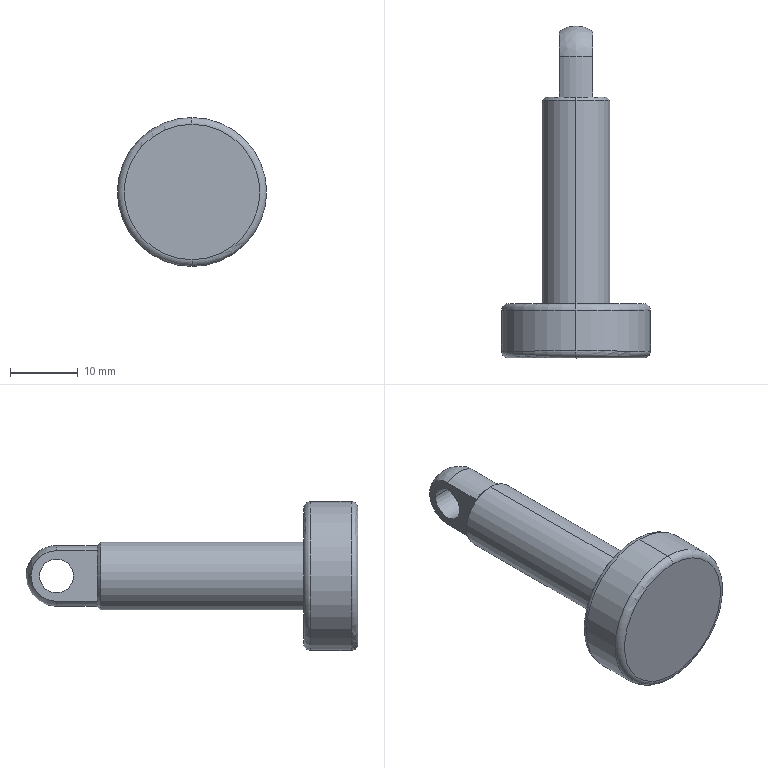Component | SolidWorks | LeverHydraulicRod22-6_HLKA-22_2-1 | 1 solid | 22 faces | box 22 x 49 x 22 mm | volume 5704 mm3 | cylinder 9 | plane 6 | torus 4 | cone 2 | sphere 1 | commonest cylinder face diameters 9 x3 22 x2 5 x2 10 x2
STEP:
#1=COLOUR_RGB('',0.7922,0.8196,0.9333);
#2=FILL_AREA_STYLE_COLOUR('',#1);
#3=FILL_AREA_STYLE('',(#2));
#4=SURFACE_STYLE_FILL_AREA(#3);
#5=SURFACE_SIDE_STYLE('',(#4));
#6=SURFACE_STYLE_USAGE(.BOTH.,#5);
#7=PRESENTATION_STYLE_ASSIGNMENT((#6));
#8=CARTESIAN_POINT('',(-2.662,2.758,4.055));
#9=VERTEX_POINT('',#8);
#10=CARTESIAN_POINT('',(-2.662,2.758,3.189));
#11=VERTEX_POINT('',#10);
#12=CARTESIAN_POINT('',(-2.662,2.758,3.622));
#13=DIRECTION('',(-0.,1.,0.));
#14=DIRECTION('',(0.,0.,-1.));
#15=AXIS2_PLACEMENT_3D('',#12,#13,#14);
#16=CIRCLE('',#15,0.4331);
#17=EDGE_CURVE('',#9,#11,#16,.T.);
#18=ORIENTED_EDGE('',*,*,#17,.F.);
#19=CARTESIAN_POINT('',(-2.662,2.718,4.016));
#20=VERTEX_POINT('',#19);
#21=CARTESIAN_POINT('',(-2.662,2.758,4.016));
#22=DIRECTION('',(1.,0.,0.));
#23=DIRECTION('',(0.,0.,-1.));
#24=AXIS2_PLACEMENT_3D('',#21,#22,#23);
#25=CIRCLE('',#24,0.03937);
#26=EDGE_CURVE('',#9,#20,#25,.T.);
#27=ORIENTED_EDGE('',*,*,#26,.T.);
#28=CARTESIAN_POINT('',(-2.662,2.718,3.228));
#29=VERTEX_POINT('',#28);
#30=CARTESIAN_POINT('',(-2.662,2.718,3.622));
#31=DIRECTION('',(0.,-1.,-0.));
#32=DIRECTION('',(0.,0.,-1.));
#33=AXIS2_PLACEMENT_3D('',#30,#31,#32);
#34=CIRCLE('',#33,0.3937);
#35=EDGE_CURVE('',#29,#20,#34,.T.);
#36=ORIENTED_EDGE('',*,*,#35,.F.);
#37=CARTESIAN_POINT('',(-2.662,2.758,3.228));
#38=DIRECTION('',(-1.,-0.,-0.));
#39=DIRECTION('',(0.,0.,1.));
#40=AXIS2_PLACEMENT_3D('',#37,#38,#39);
#41=CIRCLE('',#40,0.03937);
#42=EDGE_CURVE('',#11,#29,#41,.T.);
#43=ORIENTED_EDGE('',*,*,#42,.F.);
#44=EDGE_LOOP('',(#18,#27,#36,#43));
#45=FACE_OUTER_BOUND('',#44,.T.);
#46=CARTESIAN_POINT('',(-2.662,2.758,3.622));
#47=DIRECTION('',(0.,-1.,-0.));
#48=DIRECTION('',(0.,0.,-1.));
#49=AXIS2_PLACEMENT_3D('',#46,#47,#48);
#50=TOROIDAL_SURFACE('',#49,0.3937,0.03937);
#51=ADVANCED_FACE('',(#45),#50,.T.);
#52=CARTESIAN_POINT('',(-2.662,3.033,4.016));
#53=VERTEX_POINT('',#52);
#54=CARTESIAN_POINT('',(-2.662,3.033,3.228));
#55=VERTEX_POINT('',#54);
#56=CARTESIAN_POINT('',(-2.662,3.033,3.622));
#57=DIRECTION('',(-0.,1.,0.));
#58=DIRECTION('',(0.,0.,-1.));
#59=AXIS2_PLACEMENT_3D('',#56,#57,#58);
#60=CIRCLE('',#59,0.3937);
#61=EDGE_CURVE('',#53,#55,#60,.T.);
#62=ORIENTED_EDGE('',*,*,#61,.F.);
#63=CARTESIAN_POINT('',(-2.662,2.994,4.055));
#64=VERTEX_POINT('',#63);
#65=CARTESIAN_POINT('',(-2.662,2.994,4.016));
#66=DIRECTION('',(1.,0.,0.));
#67=DIRECTION('',(0.,0.,-1.));
#68=AXIS2_PLACEMENT_3D('',#65,#66,#67);
#69=CIRCLE('',#68,0.03937);
#70=EDGE_CURVE('',#53,#64,#69,.T.);
#71=ORIENTED_EDGE('',*,*,#70,.T.);
#72=CARTESIAN_POINT('',(-2.662,2.994,3.189));
#73=VERTEX_POINT('',#72);
#74=CARTESIAN_POINT('',(-2.662,2.994,3.622));
#75=DIRECTION('',(0.,-1.,-0.));
#76=DIRECTION('',(0.,0.,-1.));
#77=AXIS2_PLACEMENT_3D('',#74,#75,#76);
#78=CIRCLE('',#77,0.4331);
#79=EDGE_CURVE('',#73,#64,#78,.T.);
#80=ORIENTED_EDGE('',*,*,#79,.F.);
#81=CARTESIAN_POINT('',(-2.662,2.994,3.228));
#82=DIRECTION('',(-1.,-0.,-0.));
#83=DIRECTION('',(0.,0.,1.));
#84=AXIS2_PLACEMENT_3D('',#81,#82,#83);
#85=CIRCLE('',#84,0.03937);
#86=EDGE_CURVE('',#55,#73,#85,.T.);
#87=ORIENTED_EDGE('',*,*,#86,.F.);
#88=EDGE_LOOP('',(#62,#71,#80,#87));
#89=FACE_OUTER_BOUND('',#88,.T.);
#90=CARTESIAN_POINT('',(-2.662,2.994,3.622));
#91=DIRECTION('',(0.,-1.,-0.));
#92=DIRECTION('',(0.,0.,-1.));
#93=AXIS2_PLACEMENT_3D('',#90,#91,#92);
#94=TOROIDAL_SURFACE('',#93,0.3937,0.03937);
#95=ADVANCED_FACE('',(#89),#94,.T.);
#96=ORIENTED_EDGE('',*,*,#17,.T.);
#97=CARTESIAN_POINT('',(-2.662,2.718,3.189));
#98=DIRECTION('',(-0.,1.,0.));
#99=VECTOR('',#98,39.37);
#100=LINE('',#97,#99);
#101=EDGE_CURVE('',#11,#73,#100,.T.);
#102=ORIENTED_EDGE('',*,*,#101,.T.);
#103=ORIENTED_EDGE('',*,*,#79,.T.);
#104=CARTESIAN_POINT('',(-2.662,2.718,4.055));
#105=DIRECTION('',(-0.,1.,0.));
#106=VECTOR('',#105,39.37);
#107=LINE('',#104,#106);
#108=EDGE_CURVE('',#9,#64,#107,.T.);
#109=ORIENTED_EDGE('',*,*,#108,.F.);
#110=EDGE_LOOP('',(#96,#102,#103,#109));
#111=FACE_OUTER_BOUND('',#110,.T.);
#112=CARTESIAN_POINT('',(-2.662,2.718,3.622));
#113=DIRECTION('',(-0.,1.,0.));
#114=DIRECTION('',(-0.,0.,1.));
#115=AXIS2_PLACEMENT_3D('',#112,#113,#114);
#116=CYLINDRICAL_SURFACE('',#115,0.4331);
#117=ADVANCED_FACE('',(#111),#116,.T.);
#118=CARTESIAN_POINT('',(-2.564,4.569,3.622));
#119=VERTEX_POINT('',#118);
#120=CARTESIAN_POINT('',(-2.564,4.372,3.622));
#121=VERTEX_POINT('',#120);
#122=CARTESIAN_POINT('',(-2.564,4.47,3.622));
#123=DIRECTION('',(-1.,-0.,-0.));
#124=DIRECTION('',(0.,-1.,0.));
#125=AXIS2_PLACEMENT_3D('',#122,#123,#124);
#126=CIRCLE('',#125,0.09843);
#127=EDGE_CURVE('',#119,#121,#126,.T.);
#128=ORIENTED_EDGE('',*,*,#127,.F.);
#129=CARTESIAN_POINT('',(-2.761,4.569,3.622));
#130=VERTEX_POINT('',#129);
#131=CARTESIAN_POINT('',(-2.465,4.569,3.622));
#132=DIRECTION('',(-1.,-0.,-0.));
#133=VECTOR('',#132,39.37);
#134=LINE('',#131,#133);
#135=EDGE_CURVE('',#119,#130,#134,.T.);
#136=ORIENTED_EDGE('',*,*,#135,.T.);
#137=CARTESIAN_POINT('',(-2.761,4.372,3.622));
#138=VERTEX_POINT('',#137);
#139=CARTESIAN_POINT('',(-2.761,4.47,3.622));
#140=DIRECTION('',(-1.,-0.,-0.));
#141=DIRECTION('',(0.,-1.,0.));
#142=AXIS2_PLACEMENT_3D('',#139,#140,#141);
#143=CIRCLE('',#142,0.09843);
#144=EDGE_CURVE('',#130,#138,#143,.T.);
#145=ORIENTED_EDGE('',*,*,#144,.T.);
#146=CARTESIAN_POINT('',(-2.465,4.372,3.622));
#147=DIRECTION('',(-1.,-0.,-0.));
#148=VECTOR('',#147,39.37);
#149=LINE('',#146,#148);
#150=EDGE_CURVE('',#121,#138,#149,.T.);
#151=ORIENTED_EDGE('',*,*,#150,.F.);
#152=EDGE_LOOP('',(#128,#136,#145,#151));
#153=FACE_OUTER_BOUND('',#152,.T.);
#154=CARTESIAN_POINT('',(-2.465,4.47,3.622));
#155=DIRECTION('',(-1.,-0.,-0.));
#156=DIRECTION('',(0.,-1.,0.));
#157=AXIS2_PLACEMENT_3D('',#154,#155,#156);
#158=CYLINDRICAL_SURFACE('',#157,0.09843);
#159=ADVANCED_FACE('',(#153),#158,.F.);
#160=CARTESIAN_POINT('',(-2.662,4.234,3.799));
#161=VERTEX_POINT('',#160);
#162=CARTESIAN_POINT('',(-2.564,4.234,3.769));
#163=VERTEX_POINT('',#162);
#164=CARTESIAN_POINT('',(-2.662,4.234,3.622));
#165=DIRECTION('',(-0.,1.,0.));
#166=DIRECTION('',(-0.,0.,1.));
#167=AXIS2_PLACEMENT_3D('',#164,#165,#166);
#168=CIRCLE('',#167,0.1772);
#169=EDGE_CURVE('',#161,#163,#168,.T.);
#170=ORIENTED_EDGE('',*,*,#169,.F.);
#171=CARTESIAN_POINT('',(-2.662,4.214,3.819));
#172=VERTEX_POINT('',#171);
#173=CARTESIAN_POINT('',(-2.662,4.234,3.799));
#174=DIRECTION('',(-0.,-0.7071,0.7071));
#175=VECTOR('',#174,39.37);
#176=LINE('',#173,#175);
#177=EDGE_CURVE('',#161,#172,#176,.T.);
#178=ORIENTED_EDGE('',*,*,#177,.T.);
#179=CARTESIAN_POINT('',(-2.662,4.214,3.425));
#180=VERTEX_POINT('',#179);
#181=CARTESIAN_POINT('',(-2.662,4.214,3.622));
#182=DIRECTION('',(0.,-1.,-0.));
#183=DIRECTION('',(-0.,0.,1.));
#184=AXIS2_PLACEMENT_3D('',#181,#182,#183);
#185=CIRCLE('',#184,0.1969);
#186=EDGE_CURVE('',#180,#172,#185,.T.);
#187=ORIENTED_EDGE('',*,*,#186,.F.);
#188=CARTESIAN_POINT('',(-2.662,4.234,3.445));
#189=VERTEX_POINT('',#188);
#190=CARTESIAN_POINT('',(-2.662,4.234,3.445));
#191=DIRECTION('',(0.,-0.7071,-0.7071));
#192=VECTOR('',#191,39.37);
#193=LINE('',#190,#192);
#194=EDGE_CURVE('',#189,#180,#193,.T.);
#195=ORIENTED_EDGE('',*,*,#194,.F.);
#196=CARTESIAN_POINT('',(-2.564,4.234,3.475));
#197=VERTEX_POINT('',#196);
#198=CARTESIAN_POINT('',(-2.662,4.234,3.622));
#199=DIRECTION('',(-0.,1.,0.));
#200=DIRECTION('',(-0.,0.,1.));
#201=AXIS2_PLACEMENT_3D('',#198,#199,#200);
#202=CIRCLE('',#201,0.1772);
#203=EDGE_CURVE('',#197,#189,#202,.T.);
#204=ORIENTED_EDGE('',*,*,#203,.F.);
#205=CARTESIAN_POINT('',(-2.662,4.234,3.622));
#206=DIRECTION('',(-0.,1.,0.));
#207=DIRECTION('',(-0.,0.,1.));
#208=AXIS2_PLACEMENT_3D('',#205,#206,#207);
#209=CIRCLE('',#208,0.1772);
#210=EDGE_CURVE('',#163,#197,#209,.T.);
#211=ORIENTED_EDGE('',*,*,#210,.F.);
#212=EDGE_LOOP('',(#170,#178,#187,#195,#204,#211));
#213=FACE_OUTER_BOUND('',#212,.T.);
#214=CARTESIAN_POINT('',(-2.662,4.234,3.622));
#215=DIRECTION('',(0.,-1.,-0.));
#216=DIRECTION('',(0.,0.,-1.));
#217=AXIS2_PLACEMENT_3D('',#214,#215,#216);
#218=CONICAL_SURFACE('',#217,0.1772,0.7854);
#219=ADVANCED_FACE('',(#213),#218,.T.);
#220=ORIENTED_EDGE('',*,*,#186,.T.);
#221=CARTESIAN_POINT('',(-2.662,3.033,3.819));
#222=VERTEX_POINT('',#221);
#223=CARTESIAN_POINT('',(-2.662,4.234,3.819));
#224=DIRECTION('',(0.,-1.,-0.));
#225=VECTOR('',#224,39.37);
#226=LINE('',#223,#225);
#227=EDGE_CURVE('',#172,#222,#226,.T.);
#228=ORIENTED_EDGE('',*,*,#227,.T.);
#229=CARTESIAN_POINT('',(-2.662,3.033,3.425));
#230=VERTEX_POINT('',#229);
#231=CARTESIAN_POINT('',(-2.662,3.033,3.622));
#232=DIRECTION('',(0.,-1.,-0.));
#233=DIRECTION('',(0.,0.,-1.));
#234=AXIS2_PLACEMENT_3D('',#231,#232,#233);
#235=CIRCLE('',#234,0.1969);
#236=EDGE_CURVE('',#230,#222,#235,.T.);
#237=ORIENTED_EDGE('',*,*,#236,.F.);
#238=CARTESIAN_POINT('',(-2.662,4.234,3.425));
#239=DIRECTION('',(0.,-1.,-0.));
#240=VECTOR('',#239,39.37);
#241=LINE('',#238,#240);
#242=EDGE_CURVE('',#180,#230,#241,.T.);
#243=ORIENTED_EDGE('',*,*,#242,.F.);
#244=EDGE_LOOP('',(#220,#228,#237,#243));
#245=FACE_OUTER_BOUND('',#244,.T.);
#246=CARTESIAN_POINT('',(-2.662,4.234,3.622));
#247=DIRECTION('',(0.,-1.,-0.));
#248=DIRECTION('',(0.,0.,-1.));
#249=AXIS2_PLACEMENT_3D('',#246,#247,#248);
#250=CYLINDRICAL_SURFACE('',#249,0.1969);
#251=ADVANCED_FACE('',(#245),#250,.T.);
#252=CARTESIAN_POINT('',(-2.662,4.47,3.445));
#253=VERTEX_POINT('',#252);
#254=CARTESIAN_POINT('',(-2.761,4.47,3.475));
#255=VERTEX_POINT('',#254);
#256=CARTESIAN_POINT('',(-2.662,4.47,3.622));
#257=DIRECTION('',(-0.,1.,0.));
#258=DIRECTION('',(-0.,0.,1.));
#259=AXIS2_PLACEMENT_3D('',#256,#257,#258);
#260=CIRCLE('',#259,0.1772);
#261=EDGE_CURVE('',#253,#255,#260,.T.);
#262=ORIENTED_EDGE('',*,*,#261,.F.);
#263=CARTESIAN_POINT('',(-2.662,4.648,3.445));
#264=DIRECTION('',(0.,-1.,-0.));
#265=VECTOR('',#264,39.37);
#266=LINE('',#263,#265);
#267=EDGE_CURVE('',#253,#189,#266,.T.);
#268=ORIENTED_EDGE('',*,*,#267,.T.);
#269=CARTESIAN_POINT('',(-2.761,4.234,3.475));
#270=VERTEX_POINT('',#269);
#271=CARTESIAN_POINT('',(-2.662,4.234,3.622));
#272=DIRECTION('',(-0.,1.,0.));
#273=DIRECTION('',(-0.,0.,1.));
#274=AXIS2_PLACEMENT_3D('',#271,#272,#273);
#275=CIRCLE('',#274,0.1772);
#276=EDGE_CURVE('',#189,#270,#275,.T.);
#277=ORIENTED_EDGE('',*,*,#276,.T.);
#278=CARTESIAN_POINT('',(-2.761,4.648,3.475));
#279=DIRECTION('',(0.,-1.,-0.));
#280=VECTOR('',#279,39.37);
#281=LINE('',#278,#280);
#282=EDGE_CURVE('',#255,#270,#281,.T.);
#283=ORIENTED_EDGE('',*,*,#282,.F.);
#284=EDGE_LOOP('',(#262,#268,#277,#283));
#285=FACE_OUTER_BOUND('',#284,.T.);
#286=CARTESIAN_POINT('',(-2.662,4.648,3.622));
#287=DIRECTION('',(0.,-1.,-0.));
#288=DIRECTION('',(0.,0.,-1.));
#289=AXIS2_PLACEMENT_3D('',#286,#287,#288);
#290=CYLINDRICAL_SURFACE('',#289,0.1772);
#291=ADVANCED_FACE('',(#285),#290,.T.);
#292=ORIENTED_EDGE('',*,*,#35,.T.);
#293=CARTESIAN_POINT('',(-2.662,2.718,3.622));
#294=DIRECTION('',(0.,-1.,-0.));
#295=DIRECTION('',(0.,0.,-1.));
#296=AXIS2_PLACEMENT_3D('',#293,#294,#295);
#297=CIRCLE('',#296,0.3937);
#298=EDGE_CURVE('',#20,#29,#297,.T.);
#299=ORIENTED_EDGE('',*,*,#298,.T.);
#300=EDGE_LOOP('',(#292,#299));
#301=FACE_OUTER_BOUND('',#300,.T.);
#302=CARTESIAN_POINT('',(-2.662,2.718,3.622));
#303=DIRECTION('',(0.,-1.,-0.));
#304=DIRECTION('',(-1.,-0.,-0.));
#305=AXIS2_PLACEMENT_3D('',#302,#303,#304);
#306=PLANE('',#305);
#307=ADVANCED_FACE('',(#301),#306,.T.);
#308=ORIENTED_EDGE('',*,*,#236,.T.);
#309=CARTESIAN_POINT('',(-2.662,3.033,3.622));
#310=DIRECTION('',(0.,-1.,-0.));
#311=DIRECTION('',(0.,0.,-1.));
#312=AXIS2_PLACEMENT_3D('',#309,#310,#311);
#313=CIRCLE('',#312,0.1969);
#314=EDGE_CURVE('',#222,#230,#313,.T.);
#315=ORIENTED_EDGE('',*,*,#314,.T.);
#316=EDGE_LOOP('',(#308,#315));
#317=FACE_BOUND('',#316,.T.);
#318=CARTESIAN_POINT('',(-2.662,3.033,3.622));
#319=DIRECTION('',(-0.,1.,0.));
#320=DIRECTION('',(0.,0.,-1.));
#321=AXIS2_PLACEMENT_3D('',#318,#319,#320);
#322=CIRCLE('',#321,0.3937);
#323=EDGE_CURVE('',#55,#53,#322,.T.);
#324=ORIENTED_EDGE('',*,*,#323,.T.);
#325=ORIENTED_EDGE('',*,*,#61,.T.);
#326=EDGE_LOOP('',(#324,#325));
#327=FACE_OUTER_BOUND('',#326,.T.);
#328=CARTESIAN_POINT('',(-2.662,3.033,3.622));
#329=DIRECTION('',(0.,-1.,-0.));
#330=DIRECTION('',(-1.,-0.,-0.));
#331=AXIS2_PLACEMENT_3D('',#328,#329,#330);
#332=PLANE('',#331);
#333=ADVANCED_FACE('',(#317,#327),#332,.F.);
#334=CARTESIAN_POINT('',(-2.564,4.234,3.475));
#335=DIRECTION('',(0.,0.,-1.));
#336=VECTOR('',#335,39.37);
#337=LINE('',#334,#336);
#338=EDGE_CURVE('',#163,#197,#337,.T.);
#339=ORIENTED_EDGE('',*,*,#338,.F.);
#340=ORIENTED_EDGE('',*,*,#210,.T.);
#341=EDGE_LOOP('',(#339,#340));
#342=FACE_OUTER_BOUND('',#341,.T.);
#343=CARTESIAN_POINT('',(-2.662,4.234,3.622));
#344=DIRECTION('',(-0.,1.,0.));
#345=DIRECTION('',(-0.,-0.,1.));
#346=AXIS2_PLACEMENT_3D('',#343,#344,#345);
#347=PLANE('',#346);
#348=ADVANCED_FACE('',(#342),#347,.T.);
#349=CARTESIAN_POINT('',(-2.761,4.234,3.769));
#350=VERTEX_POINT('',#349);
#351=CARTESIAN_POINT('',(-2.761,4.234,3.475));
#352=DIRECTION('',(-0.,-0.,1.));
#353=VECTOR('',#352,39.37);
#354=LINE('',#351,#353);
#355=EDGE_CURVE('',#270,#350,#354,.T.);
#356=ORIENTED_EDGE('',*,*,#355,.F.);
#357=CARTESIAN_POINT('',(-2.662,4.234,3.622));
#358=DIRECTION('',(-0.,1.,0.));
#359=DIRECTION('',(-0.,0.,1.));
#360=AXIS2_PLACEMENT_3D('',#357,#358,#359);
#361=CIRCLE('',#360,0.1772);
#362=EDGE_CURVE('',#270,#350,#361,.T.);
#363=ORIENTED_EDGE('',*,*,#362,.T.);
#364=EDGE_LOOP('',(#356,#363));
#365=FACE_OUTER_BOUND('',#364,.T.);
#366=CARTESIAN_POINT('',(-2.662,4.234,3.622));
#367=DIRECTION('',(-0.,1.,0.));
#368=DIRECTION('',(-0.,-0.,1.));
#369=AXIS2_PLACEMENT_3D('',#366,#367,#368);
#370=PLANE('',#369);
#371=ADVANCED_FACE('',(#365),#370,.T.);
#372=CARTESIAN_POINT('',(-2.761,4.47,3.622));
#373=DIRECTION('',(-1.,-0.,-0.));
#374=DIRECTION('',(0.,-1.,0.));
#375=AXIS2_PLACEMENT_3D('',#372,#373,#374);
#376=CIRCLE('',#375,0.09843);
#377=EDGE_CURVE('',#138,#130,#376,.T.);
#378=ORIENTED_EDGE('',*,*,#377,.F.);
#379=ORIENTED_EDGE('',*,*,#144,.F.);
#380=EDGE_LOOP('',(#378,#379));
#381=FACE_BOUND('',#380,.T.);
#382=CARTESIAN_POINT('',(-2.761,4.47,3.769));
#383=VERTEX_POINT('',#382);
#384=CARTESIAN_POINT('',(-2.761,4.47,3.622));
#385=DIRECTION('',(1.,0.,0.));
#386=DIRECTION('',(0.,1.,0.));
#387=AXIS2_PLACEMENT_3D('',#384,#385,#386);
#388=CIRCLE('',#387,0.1473);
#389=EDGE_CURVE('',#255,#383,#388,.T.);
#390=ORIENTED_EDGE('',*,*,#389,.F.);
#391=ORIENTED_EDGE('',*,*,#282,.T.);
#392=ORIENTED_EDGE('',*,*,#355,.T.);
#393=CARTESIAN_POINT('',(-2.761,4.648,3.769));
#394=DIRECTION('',(0.,-1.,-0.));
#395=VECTOR('',#394,39.37);
#396=LINE('',#393,#395);
#397=EDGE_CURVE('',#383,#350,#396,.T.);
#398=ORIENTED_EDGE('',*,*,#397,.F.);
#399=EDGE_LOOP('',(#390,#391,#392,#398));
#400=FACE_OUTER_BOUND('',#399,.T.);
#401=CARTESIAN_POINT('',(-2.761,4.648,3.475));
#402=DIRECTION('',(1.,0.,0.));
#403=DIRECTION('',(-0.,-0.,1.));
#404=AXIS2_PLACEMENT_3D('',#401,#402,#403);
#405=PLANE('',#404);
#406=ADVANCED_FACE('',(#381,#400),#405,.F.);
#407=CARTESIAN_POINT('',(-2.564,4.47,3.622));
#408=DIRECTION('',(-1.,-0.,-0.));
#409=DIRECTION('',(0.,-1.,0.));
#410=AXIS2_PLACEMENT_3D('',#407,#408,#409);
#411=CIRCLE('',#410,0.09843);
#412=EDGE_CURVE('',#121,#119,#411,.T.);
#413=ORIENTED_EDGE('',*,*,#412,.T.);
#414=ORIENTED_EDGE('',*,*,#127,.T.);
#415=EDGE_LOOP('',(#413,#414));
#416=FACE_BOUND('',#415,.T.);
#417=CARTESIAN_POINT('',(-2.564,4.47,3.769));
#418=VERTEX_POINT('',#417);
#419=CARTESIAN_POINT('',(-2.564,4.47,3.475));
#420=VERTEX_POINT('',#419);
#421=CARTESIAN_POINT('',(-2.564,4.47,3.622));
#422=DIRECTION('',(-1.,-0.,-0.));
#423=DIRECTION('',(0.,-1.,0.));
#424=AXIS2_PLACEMENT_3D('',#421,#422,#423);
#425=CIRCLE('',#424,0.1473);
#426=EDGE_CURVE('',#418,#420,#425,.T.);
#427=ORIENTED_EDGE('',*,*,#426,.F.);
#428=CARTESIAN_POINT('',(-2.564,4.648,3.769));
#429=DIRECTION('',(0.,-1.,-0.));
#430=VECTOR('',#429,39.37);
#431=LINE('',#428,#430);
#432=EDGE_CURVE('',#418,#163,#431,.T.);
#433=ORIENTED_EDGE('',*,*,#432,.T.);
#434=ORIENTED_EDGE('',*,*,#338,.T.);
#435=CARTESIAN_POINT('',(-2.564,4.648,3.475));
#436=DIRECTION('',(0.,-1.,-0.));
#437=VECTOR('',#436,39.37);
#438=LINE('',#435,#437);
#439=EDGE_CURVE('',#420,#197,#438,.T.);
#440=ORIENTED_EDGE('',*,*,#439,.F.);
#441=EDGE_LOOP('',(#427,#433,#434,#440));
#442=FACE_OUTER_BOUND('',#441,.T.);
#443=CARTESIAN_POINT('',(-2.564,4.648,3.475));
#444=DIRECTION('',(-1.,-0.,-0.));
#445=DIRECTION('',(0.,-1.,-0.));
#446=AXIS2_PLACEMENT_3D('',#443,#444,#445);
#447=PLANE('',#446);
#448=ADVANCED_FACE('',(#416,#442),#447,.F.);
#449=CARTESIAN_POINT('',(-2.662,4.47,3.622));
#450=DIRECTION('',(-0.,1.,0.));
#451=DIRECTION('',(-0.,0.,1.));
#452=AXIS2_PLACEMENT_3D('',#449,#450,#451);
#453=CIRCLE('',#452,0.1772);
#454=EDGE_CURVE('',#383,#418,#453,.T.);
#455=ORIENTED_EDGE('',*,*,#454,.F.);
#456=ORIENTED_EDGE('',*,*,#397,.T.);
#457=CARTESIAN_POINT('',(-2.662,4.234,3.622));
#458=DIRECTION('',(-0.,1.,0.));
#459=DIRECTION('',(-0.,0.,1.));
#460=AXIS2_PLACEMENT_3D('',#457,#458,#459);
#461=CIRCLE('',#460,0.1772);
#462=EDGE_CURVE('',#350,#161,#461,.T.);
#463=ORIENTED_EDGE('',*,*,#462,.T.);
#464=ORIENTED_EDGE('',*,*,#169,.T.);
#465=ORIENTED_EDGE('',*,*,#432,.F.);
#466=EDGE_LOOP('',(#455,#456,#463,#464,#465));
#467=FACE_OUTER_BOUND('',#466,.T.);
#468=CARTESIAN_POINT('',(-2.662,4.648,3.622));
#469=DIRECTION('',(0.,-1.,-0.));
#470=DIRECTION('',(0.,0.,-1.));
#471=AXIS2_PLACEMENT_3D('',#468,#469,#470);
#472=CYLINDRICAL_SURFACE('',#471,0.1772);
#473=ADVANCED_FACE('',(#467),#472,.T.);
#474=ORIENTED_EDGE('',*,*,#267,.F.);
#475=CARTESIAN_POINT('',(-2.662,4.47,3.622));
#476=DIRECTION('',(-0.,1.,0.));
#477=DIRECTION('',(-0.,0.,1.));
#478=AXIS2_PLACEMENT_3D('',#475,#476,#477);
#479=CIRCLE('',#478,0.1772);
#480=EDGE_CURVE('',#420,#253,#479,.T.);
#481=ORIENTED_EDGE('',*,*,#480,.F.);
#482=ORIENTED_EDGE('',*,*,#439,.T.);
#483=ORIENTED_EDGE('',*,*,#203,.T.);
#484=EDGE_LOOP('',(#474,#481,#482,#483));
#485=FACE_OUTER_BOUND('',#484,.T.);
#486=CARTESIAN_POINT('',(-2.662,4.648,3.622));
#487=DIRECTION('',(0.,-1.,-0.));
#488=DIRECTION('',(0.,0.,-1.));
#489=AXIS2_PLACEMENT_3D('',#486,#487,#488);
#490=CYLINDRICAL_SURFACE('',#489,0.1772);
#491=ADVANCED_FACE('',(#485),#490,.T.);
#492=ORIENTED_EDGE('',*,*,#227,.F.);
#493=CARTESIAN_POINT('',(-2.662,4.214,3.622));
#494=DIRECTION('',(0.,-1.,-0.));
#495=DIRECTION('',(-0.,0.,1.));
#496=AXIS2_PLACEMENT_3D('',#493,#494,#495);
#497=CIRCLE('',#496,0.1969);
#498=EDGE_CURVE('',#172,#180,#497,.T.);
#499=ORIENTED_EDGE('',*,*,#498,.T.);
#500=ORIENTED_EDGE('',*,*,#242,.T.);
#501=ORIENTED_EDGE('',*,*,#314,.F.);
#502=EDGE_LOOP('',(#492,#499,#500,#501));
#503=FACE_OUTER_BOUND('',#502,.T.);
#504=CARTESIAN_POINT('',(-2.662,4.234,3.622));
#505=DIRECTION('',(0.,-1.,-0.));
#506=DIRECTION('',(0.,0.,-1.));
#507=AXIS2_PLACEMENT_3D('',#504,#505,#506);
#508=CYLINDRICAL_SURFACE('',#507,0.1969);
#509=ADVANCED_FACE('',(#503),#508,.T.);
#510=ORIENTED_EDGE('',*,*,#177,.F.);
#511=ORIENTED_EDGE('',*,*,#462,.F.);
#512=ORIENTED_EDGE('',*,*,#362,.F.);
#513=ORIENTED_EDGE('',*,*,#276,.F.);
#514=ORIENTED_EDGE('',*,*,#194,.T.);
#515=ORIENTED_EDGE('',*,*,#498,.F.);
#516=EDGE_LOOP('',(#510,#511,#512,#513,#514,#515));
#517=FACE_OUTER_BOUND('',#516,.T.);
#518=CARTESIAN_POINT('',(-2.662,4.234,3.622));
#519=DIRECTION('',(0.,-1.,-0.));
#520=DIRECTION('',(0.,0.,-1.));
#521=AXIS2_PLACEMENT_3D('',#518,#519,#520);
#522=CONICAL_SURFACE('',#521,0.1772,0.7854);
#523=ADVANCED_FACE('',(#517),#522,.T.);
#524=ORIENTED_EDGE('',*,*,#135,.F.);
#525=ORIENTED_EDGE('',*,*,#412,.F.);
#526=ORIENTED_EDGE('',*,*,#150,.T.);
#527=ORIENTED_EDGE('',*,*,#377,.T.);
#528=EDGE_LOOP('',(#524,#525,#526,#527));
#529=FACE_OUTER_BOUND('',#528,.T.);
#530=CARTESIAN_POINT('',(-2.465,4.47,3.622));
#531=DIRECTION('',(-1.,-0.,-0.));
#532=DIRECTION('',(0.,-1.,0.));
#533=AXIS2_PLACEMENT_3D('',#530,#531,#532);
#534=CYLINDRICAL_SURFACE('',#533,0.09843);
#535=ADVANCED_FACE('',(#529),#534,.F.);
#536=ORIENTED_EDGE('',*,*,#480,.T.);
#537=ORIENTED_EDGE('',*,*,#261,.T.);
#538=ORIENTED_EDGE('',*,*,#389,.T.);
#539=ORIENTED_EDGE('',*,*,#454,.T.);
#540=ORIENTED_EDGE('',*,*,#426,.T.);
#541=EDGE_LOOP('',(#536,#537,#538,#539,#540));
#542=FACE_OUTER_BOUND('',#541,.T.);
#543=CARTESIAN_POINT('',(-2.662,4.47,3.622));
#544=DIRECTION('',(0.,-1.,0.));
#545=DIRECTION('',(-0.,0.,1.));
#546=AXIS2_PLACEMENT_3D('',#543,#544,#545);
#547=SPHERICAL_SURFACE('',#546,0.1772);
#548=ADVANCED_FACE('',(#542),#547,.T.);
#549=ORIENTED_EDGE('',*,*,#101,.F.);
#550=CARTESIAN_POINT('',(-2.662,2.758,3.622));
#551=DIRECTION('',(-0.,1.,0.));
#552=DIRECTION('',(0.,0.,-1.));
#553=AXIS2_PLACEMENT_3D('',#550,#551,#552);
#554=CIRCLE('',#553,0.4331);
#555=EDGE_CURVE('',#11,#9,#554,.T.);
#556=ORIENTED_EDGE('',*,*,#555,.T.);
#557=ORIENTED_EDGE('',*,*,#108,.T.);
#558=CARTESIAN_POINT('',(-2.662,2.994,3.622));
#559=DIRECTION('',(0.,-1.,-0.));
#560=DIRECTION('',(0.,0.,-1.));
#561=AXIS2_PLACEMENT_3D('',#558,#559,#560);
#562=CIRCLE('',#561,0.4331);
#563=EDGE_CURVE('',#64,#73,#562,.T.);
#564=ORIENTED_EDGE('',*,*,#563,.T.);
#565=EDGE_LOOP('',(#549,#556,#557,#564));
#566=FACE_OUTER_BOUND('',#565,.T.);
#567=CARTESIAN_POINT('',(-2.662,2.718,3.622));
#568=DIRECTION('',(-0.,1.,0.));
#569=DIRECTION('',(-0.,0.,1.));
#570=AXIS2_PLACEMENT_3D('',#567,#568,#569);
#571=CYLINDRICAL_SURFACE('',#570,0.4331);
#572=ADVANCED_FACE('',(#566),#571,.T.);
#573=ORIENTED_EDGE('',*,*,#70,.F.);
#574=ORIENTED_EDGE('',*,*,#323,.F.);
#575=ORIENTED_EDGE('',*,*,#86,.T.);
#576=ORIENTED_EDGE('',*,*,#563,.F.);
#577=EDGE_LOOP('',(#573,#574,#575,#576));
#578=FACE_OUTER_BOUND('',#577,.T.);
#579=CARTESIAN_POINT('',(-2.662,2.994,3.622));
#580=DIRECTION('',(0.,-1.,-0.));
#581=DIRECTION('',(0.,0.,-1.));
#582=AXIS2_PLACEMENT_3D('',#579,#580,#581);
#583=TOROIDAL_SURFACE('',#582,0.3937,0.03937);
#584=ADVANCED_FACE('',(#578),#583,.T.);
#585=ORIENTED_EDGE('',*,*,#26,.F.);
#586=ORIENTED_EDGE('',*,*,#555,.F.);
#587=ORIENTED_EDGE('',*,*,#42,.T.);
#588=ORIENTED_EDGE('',*,*,#298,.F.);
#589=EDGE_LOOP('',(#585,#586,#587,#588));
#590=FACE_OUTER_BOUND('',#589,.T.);
#591=CARTESIAN_POINT('',(-2.662,2.758,3.622));
#592=DIRECTION('',(0.,-1.,-0.));
#593=DIRECTION('',(0.,0.,-1.));
#594=AXIS2_PLACEMENT_3D('',#591,#592,#593);
#595=TOROIDAL_SURFACE('',#594,0.3937,0.03937);
#596=ADVANCED_FACE('',(#590),#595,.T.);
#597=CLOSED_SHELL('',(#51,#95,#117,#159,#219,#251,#291,#307,#333,#348,#371,#406,#448,#473,#491,#509,#523,#535,#548,#572,#584,#596));
#598=MANIFOLD_SOLID_BREP('',#597);
#599=STYLED_ITEM('',(#7),#598);
#600=PRESENTATION_LAYER_ASSIGNMENT('','',(#599));
#601=CARTESIAN_POINT('',(0.,0.,0.));
#602=DIRECTION('',(0.,0.,1.));
#603=DIRECTION('',(1.,0.,0.));
#604=AXIS2_PLACEMENT_3D('',#601,#602,#603);
#605=(LENGTH_UNIT()NAMED_UNIT(*)SI_UNIT($,.METRE.));
#606=LENGTH_MEASURE_WITH_UNIT(LENGTH_MEASURE(0.0254),#605);
#607=DIMENSIONAL_EXPONENTS(1.,0.,0.,0.,0.,0.,0.);
#608=(CONVERSION_BASED_UNIT('',#606)LENGTH_UNIT()NAMED_UNIT(#607));
#609=UNCERTAINTY_MEASURE_WITH_UNIT(LENGTH_MEASURE(0.00001),#608,'','');
#610=(NAMED_UNIT(*)PLANE_ANGLE_UNIT()SI_UNIT($,.RADIAN.));
#611=(NAMED_UNIT(*)SI_UNIT($,.STERADIAN.)SOLID_ANGLE_UNIT());
#612=(GEOMETRIC_REPRESENTATION_CONTEXT(3)GLOBAL_UNCERTAINTY_ASSIGNED_CONTEXT((#609))GLOBAL_UNIT_ASSIGNED_CONTEXT((#608,#610,#611))REPRESENTATION_CONTEXT('',''));
#613=ADVANCED_BREP_SHAPE_REPRESENTATION('',(#598,#604),#612);
#614=(LENGTH_UNIT()NAMED_UNIT(*)SI_UNIT($,.METRE.));
#615=LENGTH_MEASURE_WITH_UNIT(LENGTH_MEASURE(0.0254),#614);
#616=DIMENSIONAL_EXPONENTS(1.,0.,0.,0.,0.,0.,0.);
#617=(CONVERSION_BASED_UNIT('',#615)LENGTH_UNIT()NAMED_UNIT(#616));
#618=UNCERTAINTY_MEASURE_WITH_UNIT(LENGTH_MEASURE(0.00001),#617,'','');
#619=(NAMED_UNIT(*)PLANE_ANGLE_UNIT()SI_UNIT($,.RADIAN.));
#620=(NAMED_UNIT(*)SI_UNIT($,.STERADIAN.)SOLID_ANGLE_UNIT());
#621=(GEOMETRIC_REPRESENTATION_CONTEXT(3)GLOBAL_UNCERTAINTY_ASSIGNED_CONTEXT((#618))GLOBAL_UNIT_ASSIGNED_CONTEXT((#617,#619,#620))REPRESENTATION_CONTEXT('',''));
#622=MECHANICAL_DESIGN_GEOMETRIC_PRESENTATION_REPRESENTATION('',(#599),#621);